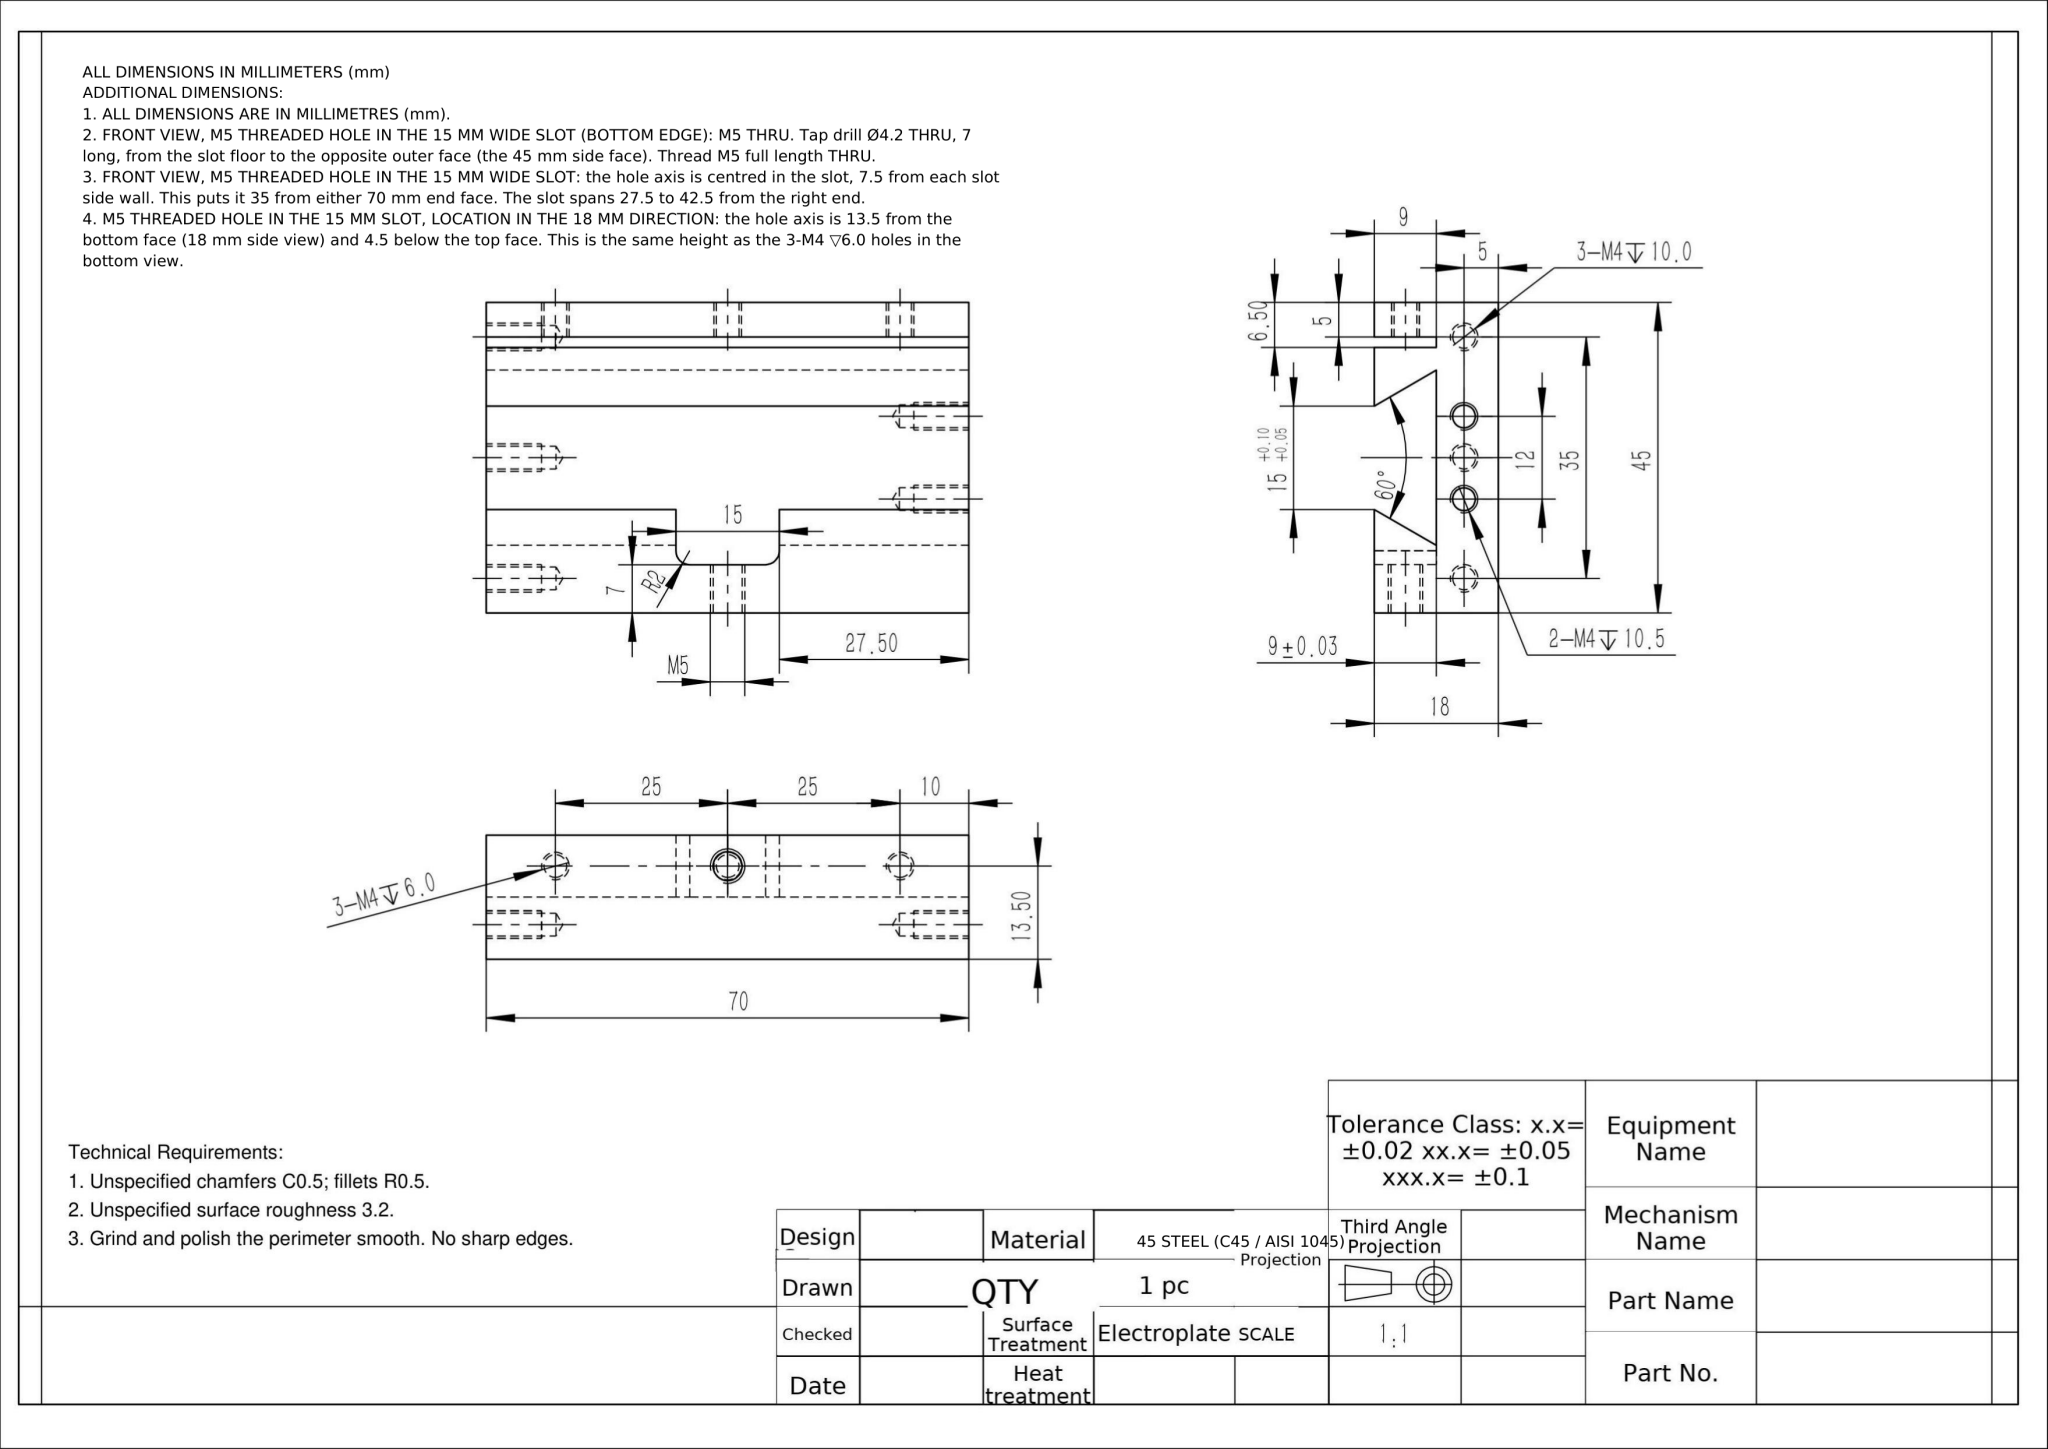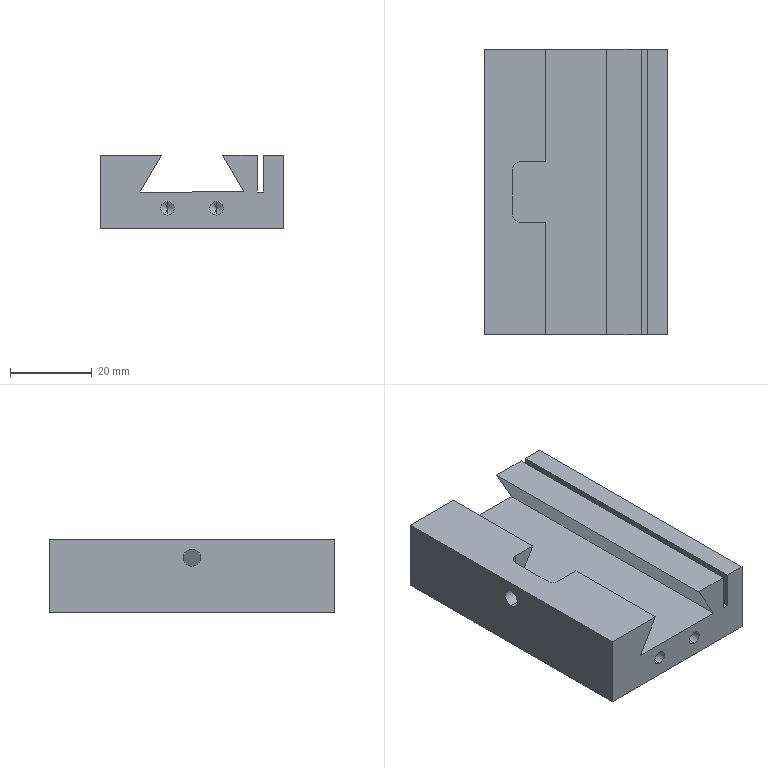Part | NX | mm | Angled Vise Jaw Block | 1 solid | 48 faces | box 45 x 70 x 18 mm | volume 41646 mm3 | cylinder 20 | plane 18 | cone 10 | commonest cylinder face diameters 3.3 x16 4.2 x2 4 x2